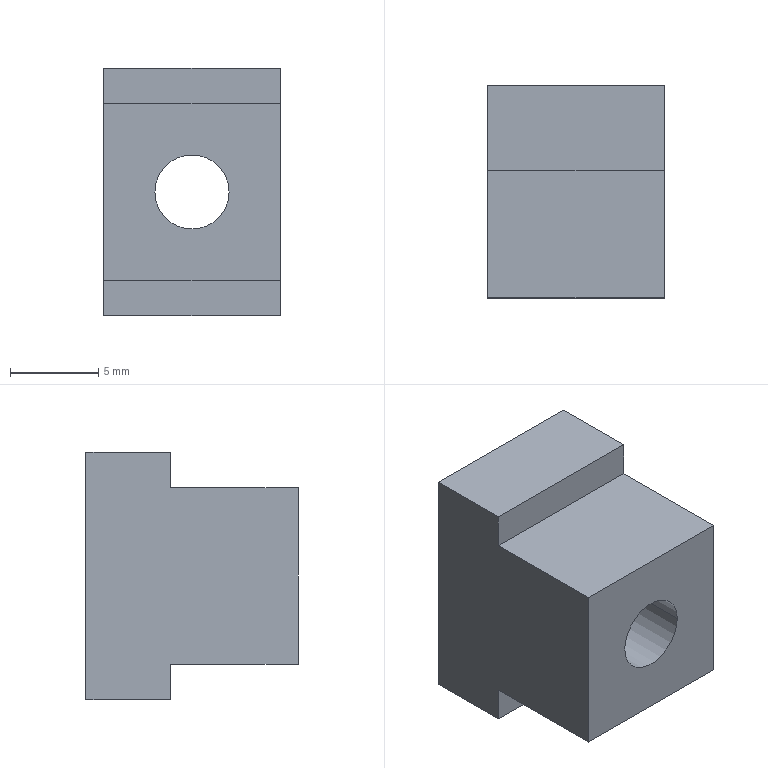Component | SolidWorks | 7.1.02.0001.00.00-0052-1 | 1 solid | 12 faces | box 10 x 12 x 14 mm | volume 1226 mm3 | plane 10 | cylinder 2 | commonest cylinder face diameters 4.2 x2
build123d program:
from build123d import *

# Parameters (mm, degrees)
BOSS_EXTRUDE1_DEPTH   = 10
M5X0_8_TAPPED_HOLE1_D = 4.2


with BuildPart() as part:
    # Sketch1 → Boss-Extrude1 (new body)
    with BuildSketch(Plane.XY):
        Polygon((-1.2, 7), (-1.2, 5), (6, 5), (6, -5), (-1.2, -5), (-1.2, -7), (-6, -7), (-6, 7), align=None)
    extrude(amount=BOSS_EXTRUDE1_DEPTH)

    # M5x0.8 Tapped Hole1 (through all)
    with Locations(Plane(origin=(6, 0, 5), x_dir=(0, 0, 1), z_dir=(1, 0, 0))):
        with Locations((0, 0)):
            Hole(M5X0_8_TAPPED_HOLE1_D / 2)


solid = part.part

# Placed as in the assembly
solid = solid.moved(Location((-49.064, -2.684, 0), (90, -90, 0)))
STEP:
#1=COLOUR_RGB('',0.7922,0.8196,0.9333);
#2=FILL_AREA_STYLE_COLOUR('',#1);
#3=FILL_AREA_STYLE('',(#2));
#4=SURFACE_STYLE_FILL_AREA(#3);
#5=SURFACE_SIDE_STYLE('',(#4));
#6=SURFACE_STYLE_USAGE(.BOTH.,#5);
#7=PRESENTATION_STYLE_ASSIGNMENT((#6));
#8=CARTESIAN_POINT('',(-2.211,0.1306,0.));
#9=VERTEX_POINT('',#8);
#10=CARTESIAN_POINT('',(-2.046,0.1306,0.));
#11=VERTEX_POINT('',#10);
#12=CARTESIAN_POINT('',(-2.128,0.1306,0.));
#13=DIRECTION('',(0.,-1.,-0.));
#14=DIRECTION('',(1.,0.,-0.));
#15=AXIS2_PLACEMENT_3D('',#12,#13,#14);
#16=CIRCLE('',#15,0.08268);
#17=EDGE_CURVE('',#9,#11,#16,.T.);
#18=ORIENTED_EDGE('',*,*,#17,.F.);
#19=CARTESIAN_POINT('',(-2.211,-0.3419,0.));
#20=VERTEX_POINT('',#19);
#21=CARTESIAN_POINT('',(-2.211,-0.3419,0.));
#22=DIRECTION('',(0.,-1.,-0.));
#23=VECTOR('',#22,39.37);
#24=LINE('',#21,#23);
#25=EDGE_CURVE('',#9,#20,#24,.T.);
#26=ORIENTED_EDGE('',*,*,#25,.T.);
#27=CARTESIAN_POINT('',(-2.046,-0.3419,0.));
#28=VERTEX_POINT('',#27);
#29=CARTESIAN_POINT('',(-2.128,-0.3419,0.));
#30=DIRECTION('',(0.,-1.,-0.));
#31=DIRECTION('',(1.,0.,-0.));
#32=AXIS2_PLACEMENT_3D('',#29,#30,#31);
#33=CIRCLE('',#32,0.08268);
#34=EDGE_CURVE('',#20,#28,#33,.T.);
#35=ORIENTED_EDGE('',*,*,#34,.T.);
#36=CARTESIAN_POINT('',(-2.046,-0.3419,0.));
#37=DIRECTION('',(0.,-1.,-0.));
#38=VECTOR('',#37,39.37);
#39=LINE('',#36,#38);
#40=EDGE_CURVE('',#11,#28,#39,.T.);
#41=ORIENTED_EDGE('',*,*,#40,.F.);
#42=EDGE_LOOP('',(#18,#26,#35,#41));
#43=FACE_OUTER_BOUND('',#42,.T.);
#44=CARTESIAN_POINT('',(-2.128,-0.3419,0.));
#45=DIRECTION('',(0.,-1.,-0.));
#46=DIRECTION('',(1.,0.,-0.));
#47=AXIS2_PLACEMENT_3D('',#44,#45,#46);
#48=CYLINDRICAL_SURFACE('',#47,0.08268);
#49=ADVANCED_FACE('',(#43),#48,.F.);
#50=CARTESIAN_POINT('',(-2.128,0.1306,0.));
#51=DIRECTION('',(0.,-1.,-0.));
#52=DIRECTION('',(1.,0.,-0.));
#53=AXIS2_PLACEMENT_3D('',#50,#51,#52);
#54=CIRCLE('',#53,0.08268);
#55=EDGE_CURVE('',#11,#9,#54,.T.);
#56=ORIENTED_EDGE('',*,*,#55,.T.);
#57=ORIENTED_EDGE('',*,*,#17,.T.);
#58=EDGE_LOOP('',(#56,#57));
#59=FACE_BOUND('',#58,.T.);
#60=CARTESIAN_POINT('',(-1.932,0.1306,0.2756));
#61=VERTEX_POINT('',#60);
#62=CARTESIAN_POINT('',(-1.932,0.1306,-0.2756));
#63=VERTEX_POINT('',#62);
#64=CARTESIAN_POINT('',(-1.932,0.1306,0.2756));
#65=DIRECTION('',(-0.,0.,-1.));
#66=VECTOR('',#65,39.37);
#67=LINE('',#64,#66);
#68=EDGE_CURVE('',#61,#63,#67,.T.);
#69=ORIENTED_EDGE('',*,*,#68,.T.);
#70=CARTESIAN_POINT('',(-2.325,0.1306,-0.2756));
#71=VERTEX_POINT('',#70);
#72=CARTESIAN_POINT('',(-2.325,0.1306,-0.2756));
#73=DIRECTION('',(1.,0.,-0.));
#74=VECTOR('',#73,39.37);
#75=LINE('',#72,#74);
#76=EDGE_CURVE('',#71,#63,#75,.T.);
#77=ORIENTED_EDGE('',*,*,#76,.F.);
#78=CARTESIAN_POINT('',(-2.325,0.1306,0.2756));
#79=VERTEX_POINT('',#78);
#80=CARTESIAN_POINT('',(-2.325,0.1306,0.2756));
#81=DIRECTION('',(-0.,0.,-1.));
#82=VECTOR('',#81,39.37);
#83=LINE('',#80,#82);
#84=EDGE_CURVE('',#79,#71,#83,.T.);
#85=ORIENTED_EDGE('',*,*,#84,.F.);
#86=CARTESIAN_POINT('',(-2.325,0.1306,0.2756));
#87=DIRECTION('',(1.,0.,-0.));
#88=VECTOR('',#87,39.37);
#89=LINE('',#86,#88);
#90=EDGE_CURVE('',#79,#61,#89,.T.);
#91=ORIENTED_EDGE('',*,*,#90,.T.);
#92=EDGE_LOOP('',(#69,#77,#85,#91));
#93=FACE_OUTER_BOUND('',#92,.T.);
#94=CARTESIAN_POINT('',(-2.325,0.1306,0.2756));
#95=DIRECTION('',(0.,-1.,-0.));
#96=DIRECTION('',(1.,0.,-0.));
#97=AXIS2_PLACEMENT_3D('',#94,#95,#96);
#98=PLANE('',#97);
#99=ADVANCED_FACE('',(#59,#93),#98,.F.);
#100=CARTESIAN_POINT('',(-1.932,-0.05842,-0.2756));
#101=VERTEX_POINT('',#100);
#102=CARTESIAN_POINT('',(-1.932,0.1306,-0.2756));
#103=DIRECTION('',(0.,-1.,-0.));
#104=VECTOR('',#103,39.37);
#105=LINE('',#102,#104);
#106=EDGE_CURVE('',#63,#101,#105,.T.);
#107=ORIENTED_EDGE('',*,*,#106,.T.);
#108=CARTESIAN_POINT('',(-2.325,-0.05842,-0.2756));
#109=VERTEX_POINT('',#108);
#110=CARTESIAN_POINT('',(-2.325,-0.05842,-0.2756));
#111=DIRECTION('',(1.,0.,-0.));
#112=VECTOR('',#111,39.37);
#113=LINE('',#110,#112);
#114=EDGE_CURVE('',#109,#101,#113,.T.);
#115=ORIENTED_EDGE('',*,*,#114,.F.);
#116=CARTESIAN_POINT('',(-2.325,0.1306,-0.2756));
#117=DIRECTION('',(0.,-1.,-0.));
#118=VECTOR('',#117,39.37);
#119=LINE('',#116,#118);
#120=EDGE_CURVE('',#71,#109,#119,.T.);
#121=ORIENTED_EDGE('',*,*,#120,.F.);
#122=ORIENTED_EDGE('',*,*,#76,.T.);
#123=EDGE_LOOP('',(#107,#115,#121,#122));
#124=FACE_OUTER_BOUND('',#123,.T.);
#125=CARTESIAN_POINT('',(-2.325,0.1306,-0.2756));
#126=DIRECTION('',(0.,-0.,1.));
#127=DIRECTION('',(-1.,-0.,0.));
#128=AXIS2_PLACEMENT_3D('',#125,#126,#127);
#129=PLANE('',#128);
#130=ADVANCED_FACE('',(#124),#129,.F.);
#131=CARTESIAN_POINT('',(-1.932,-0.05842,-0.1969));
#132=VERTEX_POINT('',#131);
#133=CARTESIAN_POINT('',(-1.932,-0.05842,-0.2756));
#134=DIRECTION('',(0.,-0.,1.));
#135=VECTOR('',#134,39.37);
#136=LINE('',#133,#135);
#137=EDGE_CURVE('',#101,#132,#136,.T.);
#138=ORIENTED_EDGE('',*,*,#137,.T.);
#139=CARTESIAN_POINT('',(-2.325,-0.05842,-0.1969));
#140=VERTEX_POINT('',#139);
#141=CARTESIAN_POINT('',(-2.325,-0.05842,-0.1969));
#142=DIRECTION('',(1.,0.,-0.));
#143=VECTOR('',#142,39.37);
#144=LINE('',#141,#143);
#145=EDGE_CURVE('',#140,#132,#144,.T.);
#146=ORIENTED_EDGE('',*,*,#145,.F.);
#147=CARTESIAN_POINT('',(-2.325,-0.05842,-0.2756));
#148=DIRECTION('',(0.,-0.,1.));
#149=VECTOR('',#148,39.37);
#150=LINE('',#147,#149);
#151=EDGE_CURVE('',#109,#140,#150,.T.);
#152=ORIENTED_EDGE('',*,*,#151,.F.);
#153=ORIENTED_EDGE('',*,*,#114,.T.);
#154=EDGE_LOOP('',(#138,#146,#152,#153));
#155=FACE_OUTER_BOUND('',#154,.T.);
#156=CARTESIAN_POINT('',(-2.325,-0.05842,-0.2756));
#157=DIRECTION('',(-0.,1.,0.));
#158=DIRECTION('',(-1.,-0.,0.));
#159=AXIS2_PLACEMENT_3D('',#156,#157,#158);
#160=PLANE('',#159);
#161=ADVANCED_FACE('',(#155),#160,.F.);
#162=CARTESIAN_POINT('',(-1.932,-0.3419,-0.1969));
#163=VERTEX_POINT('',#162);
#164=CARTESIAN_POINT('',(-1.932,-0.05842,-0.1969));
#165=DIRECTION('',(0.,-1.,-0.));
#166=VECTOR('',#165,39.37);
#167=LINE('',#164,#166);
#168=EDGE_CURVE('',#132,#163,#167,.T.);
#169=ORIENTED_EDGE('',*,*,#168,.T.);
#170=CARTESIAN_POINT('',(-2.325,-0.3419,-0.1969));
#171=VERTEX_POINT('',#170);
#172=CARTESIAN_POINT('',(-2.325,-0.3419,-0.1969));
#173=DIRECTION('',(1.,0.,-0.));
#174=VECTOR('',#173,39.37);
#175=LINE('',#172,#174);
#176=EDGE_CURVE('',#171,#163,#175,.T.);
#177=ORIENTED_EDGE('',*,*,#176,.F.);
#178=CARTESIAN_POINT('',(-2.325,-0.05842,-0.1969));
#179=DIRECTION('',(0.,-1.,-0.));
#180=VECTOR('',#179,39.37);
#181=LINE('',#178,#180);
#182=EDGE_CURVE('',#140,#171,#181,.T.);
#183=ORIENTED_EDGE('',*,*,#182,.F.);
#184=ORIENTED_EDGE('',*,*,#145,.T.);
#185=EDGE_LOOP('',(#169,#177,#183,#184));
#186=FACE_OUTER_BOUND('',#185,.T.);
#187=CARTESIAN_POINT('',(-2.325,-0.05842,-0.1969));
#188=DIRECTION('',(0.,-0.,1.));
#189=DIRECTION('',(-1.,-0.,0.));
#190=AXIS2_PLACEMENT_3D('',#187,#188,#189);
#191=PLANE('',#190);
#192=ADVANCED_FACE('',(#186),#191,.F.);
#193=CARTESIAN_POINT('',(-2.128,-0.3419,0.));
#194=DIRECTION('',(0.,-1.,-0.));
#195=DIRECTION('',(1.,0.,-0.));
#196=AXIS2_PLACEMENT_3D('',#193,#194,#195);
#197=CIRCLE('',#196,0.08268);
#198=EDGE_CURVE('',#28,#20,#197,.T.);
#199=ORIENTED_EDGE('',*,*,#198,.F.);
#200=ORIENTED_EDGE('',*,*,#34,.F.);
#201=EDGE_LOOP('',(#199,#200));
#202=FACE_BOUND('',#201,.T.);
#203=CARTESIAN_POINT('',(-1.932,-0.3419,0.1969));
#204=VERTEX_POINT('',#203);
#205=CARTESIAN_POINT('',(-1.932,-0.3419,0.1969));
#206=DIRECTION('',(0.,-0.,1.));
#207=VECTOR('',#206,39.37);
#208=LINE('',#205,#207);
#209=EDGE_CURVE('',#163,#204,#208,.T.);
#210=ORIENTED_EDGE('',*,*,#209,.T.);
#211=CARTESIAN_POINT('',(-2.325,-0.3419,0.1969));
#212=VERTEX_POINT('',#211);
#213=CARTESIAN_POINT('',(-2.325,-0.3419,0.1969));
#214=DIRECTION('',(1.,0.,-0.));
#215=VECTOR('',#214,39.37);
#216=LINE('',#213,#215);
#217=EDGE_CURVE('',#212,#204,#216,.T.);
#218=ORIENTED_EDGE('',*,*,#217,.F.);
#219=CARTESIAN_POINT('',(-2.325,-0.3419,0.1969));
#220=DIRECTION('',(0.,-0.,1.));
#221=VECTOR('',#220,39.37);
#222=LINE('',#219,#221);
#223=EDGE_CURVE('',#171,#212,#222,.T.);
#224=ORIENTED_EDGE('',*,*,#223,.F.);
#225=ORIENTED_EDGE('',*,*,#176,.T.);
#226=EDGE_LOOP('',(#210,#218,#224,#225));
#227=FACE_OUTER_BOUND('',#226,.T.);
#228=CARTESIAN_POINT('',(-2.325,-0.3419,0.1969));
#229=DIRECTION('',(-0.,1.,0.));
#230=DIRECTION('',(-1.,-0.,0.));
#231=AXIS2_PLACEMENT_3D('',#228,#229,#230);
#232=PLANE('',#231);
#233=ADVANCED_FACE('',(#202,#227),#232,.F.);
#234=CARTESIAN_POINT('',(-1.932,-0.05842,0.1969));
#235=VERTEX_POINT('',#234);
#236=CARTESIAN_POINT('',(-1.932,-0.05842,0.1969));
#237=DIRECTION('',(-0.,1.,0.));
#238=VECTOR('',#237,39.37);
#239=LINE('',#236,#238);
#240=EDGE_CURVE('',#204,#235,#239,.T.);
#241=ORIENTED_EDGE('',*,*,#240,.T.);
#242=CARTESIAN_POINT('',(-2.325,-0.05842,0.1969));
#243=VERTEX_POINT('',#242);
#244=CARTESIAN_POINT('',(-2.325,-0.05842,0.1969));
#245=DIRECTION('',(1.,0.,-0.));
#246=VECTOR('',#245,39.37);
#247=LINE('',#244,#246);
#248=EDGE_CURVE('',#243,#235,#247,.T.);
#249=ORIENTED_EDGE('',*,*,#248,.F.);
#250=CARTESIAN_POINT('',(-2.325,-0.05842,0.1969));
#251=DIRECTION('',(-0.,1.,0.));
#252=VECTOR('',#251,39.37);
#253=LINE('',#250,#252);
#254=EDGE_CURVE('',#212,#243,#253,.T.);
#255=ORIENTED_EDGE('',*,*,#254,.F.);
#256=ORIENTED_EDGE('',*,*,#217,.T.);
#257=EDGE_LOOP('',(#241,#249,#255,#256));
#258=FACE_OUTER_BOUND('',#257,.T.);
#259=CARTESIAN_POINT('',(-2.325,-0.05842,0.1969));
#260=DIRECTION('',(-0.,0.,-1.));
#261=DIRECTION('',(1.,0.,-0.));
#262=AXIS2_PLACEMENT_3D('',#259,#260,#261);
#263=PLANE('',#262);
#264=ADVANCED_FACE('',(#258),#263,.F.);
#265=CARTESIAN_POINT('',(-1.932,-0.05842,0.2756));
#266=VERTEX_POINT('',#265);
#267=CARTESIAN_POINT('',(-1.932,-0.05842,0.2756));
#268=DIRECTION('',(0.,-0.,1.));
#269=VECTOR('',#268,39.37);
#270=LINE('',#267,#269);
#271=EDGE_CURVE('',#235,#266,#270,.T.);
#272=ORIENTED_EDGE('',*,*,#271,.T.);
#273=CARTESIAN_POINT('',(-2.325,-0.05842,0.2756));
#274=VERTEX_POINT('',#273);
#275=CARTESIAN_POINT('',(-2.325,-0.05842,0.2756));
#276=DIRECTION('',(1.,0.,-0.));
#277=VECTOR('',#276,39.37);
#278=LINE('',#275,#277);
#279=EDGE_CURVE('',#274,#266,#278,.T.);
#280=ORIENTED_EDGE('',*,*,#279,.F.);
#281=CARTESIAN_POINT('',(-2.325,-0.05842,0.2756));
#282=DIRECTION('',(0.,-0.,1.));
#283=VECTOR('',#282,39.37);
#284=LINE('',#281,#283);
#285=EDGE_CURVE('',#243,#274,#284,.T.);
#286=ORIENTED_EDGE('',*,*,#285,.F.);
#287=ORIENTED_EDGE('',*,*,#248,.T.);
#288=EDGE_LOOP('',(#272,#280,#286,#287));
#289=FACE_OUTER_BOUND('',#288,.T.);
#290=CARTESIAN_POINT('',(-2.325,-0.05842,0.2756));
#291=DIRECTION('',(-0.,1.,0.));
#292=DIRECTION('',(-1.,-0.,0.));
#293=AXIS2_PLACEMENT_3D('',#290,#291,#292);
#294=PLANE('',#293);
#295=ADVANCED_FACE('',(#289),#294,.F.);
#296=CARTESIAN_POINT('',(-1.932,0.1306,0.2756));
#297=DIRECTION('',(-0.,1.,0.));
#298=VECTOR('',#297,39.37);
#299=LINE('',#296,#298);
#300=EDGE_CURVE('',#266,#61,#299,.T.);
#301=ORIENTED_EDGE('',*,*,#300,.T.);
#302=ORIENTED_EDGE('',*,*,#90,.F.);
#303=CARTESIAN_POINT('',(-2.325,0.1306,0.2756));
#304=DIRECTION('',(-0.,1.,0.));
#305=VECTOR('',#304,39.37);
#306=LINE('',#303,#305);
#307=EDGE_CURVE('',#274,#79,#306,.T.);
#308=ORIENTED_EDGE('',*,*,#307,.F.);
#309=ORIENTED_EDGE('',*,*,#279,.T.);
#310=EDGE_LOOP('',(#301,#302,#308,#309));
#311=FACE_OUTER_BOUND('',#310,.T.);
#312=CARTESIAN_POINT('',(-2.325,0.1306,0.2756));
#313=DIRECTION('',(-0.,0.,-1.));
#314=DIRECTION('',(1.,0.,-0.));
#315=AXIS2_PLACEMENT_3D('',#312,#313,#314);
#316=PLANE('',#315);
#317=ADVANCED_FACE('',(#311),#316,.F.);
#318=ORIENTED_EDGE('',*,*,#84,.T.);
#319=ORIENTED_EDGE('',*,*,#120,.T.);
#320=ORIENTED_EDGE('',*,*,#151,.T.);
#321=ORIENTED_EDGE('',*,*,#182,.T.);
#322=ORIENTED_EDGE('',*,*,#223,.T.);
#323=ORIENTED_EDGE('',*,*,#254,.T.);
#324=ORIENTED_EDGE('',*,*,#285,.T.);
#325=ORIENTED_EDGE('',*,*,#307,.T.);
#326=EDGE_LOOP('',(#318,#319,#320,#321,#322,#323,#324,#325));
#327=FACE_OUTER_BOUND('',#326,.T.);
#328=CARTESIAN_POINT('',(-2.325,-0.1057,0.));
#329=DIRECTION('',(-1.,-0.,0.));
#330=DIRECTION('',(0.,-1.,-0.));
#331=AXIS2_PLACEMENT_3D('',#328,#329,#330);
#332=PLANE('',#331);
#333=ADVANCED_FACE('',(#327),#332,.T.);
#334=ORIENTED_EDGE('',*,*,#68,.F.);
#335=ORIENTED_EDGE('',*,*,#300,.F.);
#336=ORIENTED_EDGE('',*,*,#271,.F.);
#337=ORIENTED_EDGE('',*,*,#240,.F.);
#338=ORIENTED_EDGE('',*,*,#209,.F.);
#339=ORIENTED_EDGE('',*,*,#168,.F.);
#340=ORIENTED_EDGE('',*,*,#137,.F.);
#341=ORIENTED_EDGE('',*,*,#106,.F.);
#342=EDGE_LOOP('',(#334,#335,#336,#337,#338,#339,#340,#341));
#343=FACE_OUTER_BOUND('',#342,.T.);
#344=CARTESIAN_POINT('',(-1.932,-0.1057,0.));
#345=DIRECTION('',(-1.,-0.,0.));
#346=DIRECTION('',(0.,-1.,-0.));
#347=AXIS2_PLACEMENT_3D('',#344,#345,#346);
#348=PLANE('',#347);
#349=ADVANCED_FACE('',(#343),#348,.F.);
#350=ORIENTED_EDGE('',*,*,#25,.F.);
#351=ORIENTED_EDGE('',*,*,#55,.F.);
#352=ORIENTED_EDGE('',*,*,#40,.T.);
#353=ORIENTED_EDGE('',*,*,#198,.T.);
#354=EDGE_LOOP('',(#350,#351,#352,#353));
#355=FACE_OUTER_BOUND('',#354,.T.);
#356=CARTESIAN_POINT('',(-2.128,-0.3419,0.));
#357=DIRECTION('',(0.,-1.,-0.));
#358=DIRECTION('',(1.,0.,-0.));
#359=AXIS2_PLACEMENT_3D('',#356,#357,#358);
#360=CYLINDRICAL_SURFACE('',#359,0.08268);
#361=ADVANCED_FACE('',(#355),#360,.F.);
#362=CLOSED_SHELL('',(#49,#99,#130,#161,#192,#233,#264,#295,#317,#333,#349,#361));
#363=MANIFOLD_SOLID_BREP('',#362);
#364=STYLED_ITEM('',(#7),#363);
#365=PRESENTATION_LAYER_ASSIGNMENT('','',(#364));
#366=CARTESIAN_POINT('',(0.,0.,0.));
#367=DIRECTION('',(0.,0.,1.));
#368=DIRECTION('',(1.,0.,0.));
#369=AXIS2_PLACEMENT_3D('',#366,#367,#368);
#370=(LENGTH_UNIT()NAMED_UNIT(*)SI_UNIT($,.METRE.));
#371=LENGTH_MEASURE_WITH_UNIT(LENGTH_MEASURE(0.0254),#370);
#372=DIMENSIONAL_EXPONENTS(1.,0.,0.,0.,0.,0.,0.);
#373=(CONVERSION_BASED_UNIT('',#371)LENGTH_UNIT()NAMED_UNIT(#372));
#374=UNCERTAINTY_MEASURE_WITH_UNIT(LENGTH_MEASURE(0.00001),#373,'','');
#375=(NAMED_UNIT(*)PLANE_ANGLE_UNIT()SI_UNIT($,.RADIAN.));
#376=(NAMED_UNIT(*)SI_UNIT($,.STERADIAN.)SOLID_ANGLE_UNIT());
#377=(GEOMETRIC_REPRESENTATION_CONTEXT(3)GLOBAL_UNCERTAINTY_ASSIGNED_CONTEXT((#374))GLOBAL_UNIT_ASSIGNED_CONTEXT((#373,#375,#376))REPRESENTATION_CONTEXT('',''));
#378=ADVANCED_BREP_SHAPE_REPRESENTATION('',(#363,#369),#377);
#379=(LENGTH_UNIT()NAMED_UNIT(*)SI_UNIT($,.METRE.));
#380=LENGTH_MEASURE_WITH_UNIT(LENGTH_MEASURE(0.0254),#379);
#381=DIMENSIONAL_EXPONENTS(1.,0.,0.,0.,0.,0.,0.);
#382=(CONVERSION_BASED_UNIT('',#380)LENGTH_UNIT()NAMED_UNIT(#381));
#383=UNCERTAINTY_MEASURE_WITH_UNIT(LENGTH_MEASURE(0.00001),#382,'','');
#384=(NAMED_UNIT(*)PLANE_ANGLE_UNIT()SI_UNIT($,.RADIAN.));
#385=(NAMED_UNIT(*)SI_UNIT($,.STERADIAN.)SOLID_ANGLE_UNIT());
#386=(GEOMETRIC_REPRESENTATION_CONTEXT(3)GLOBAL_UNCERTAINTY_ASSIGNED_CONTEXT((#383))GLOBAL_UNIT_ASSIGNED_CONTEXT((#382,#384,#385))REPRESENTATION_CONTEXT('',''));
#387=MECHANICAL_DESIGN_GEOMETRIC_PRESENTATION_REPRESENTATION('',(#364),#386);